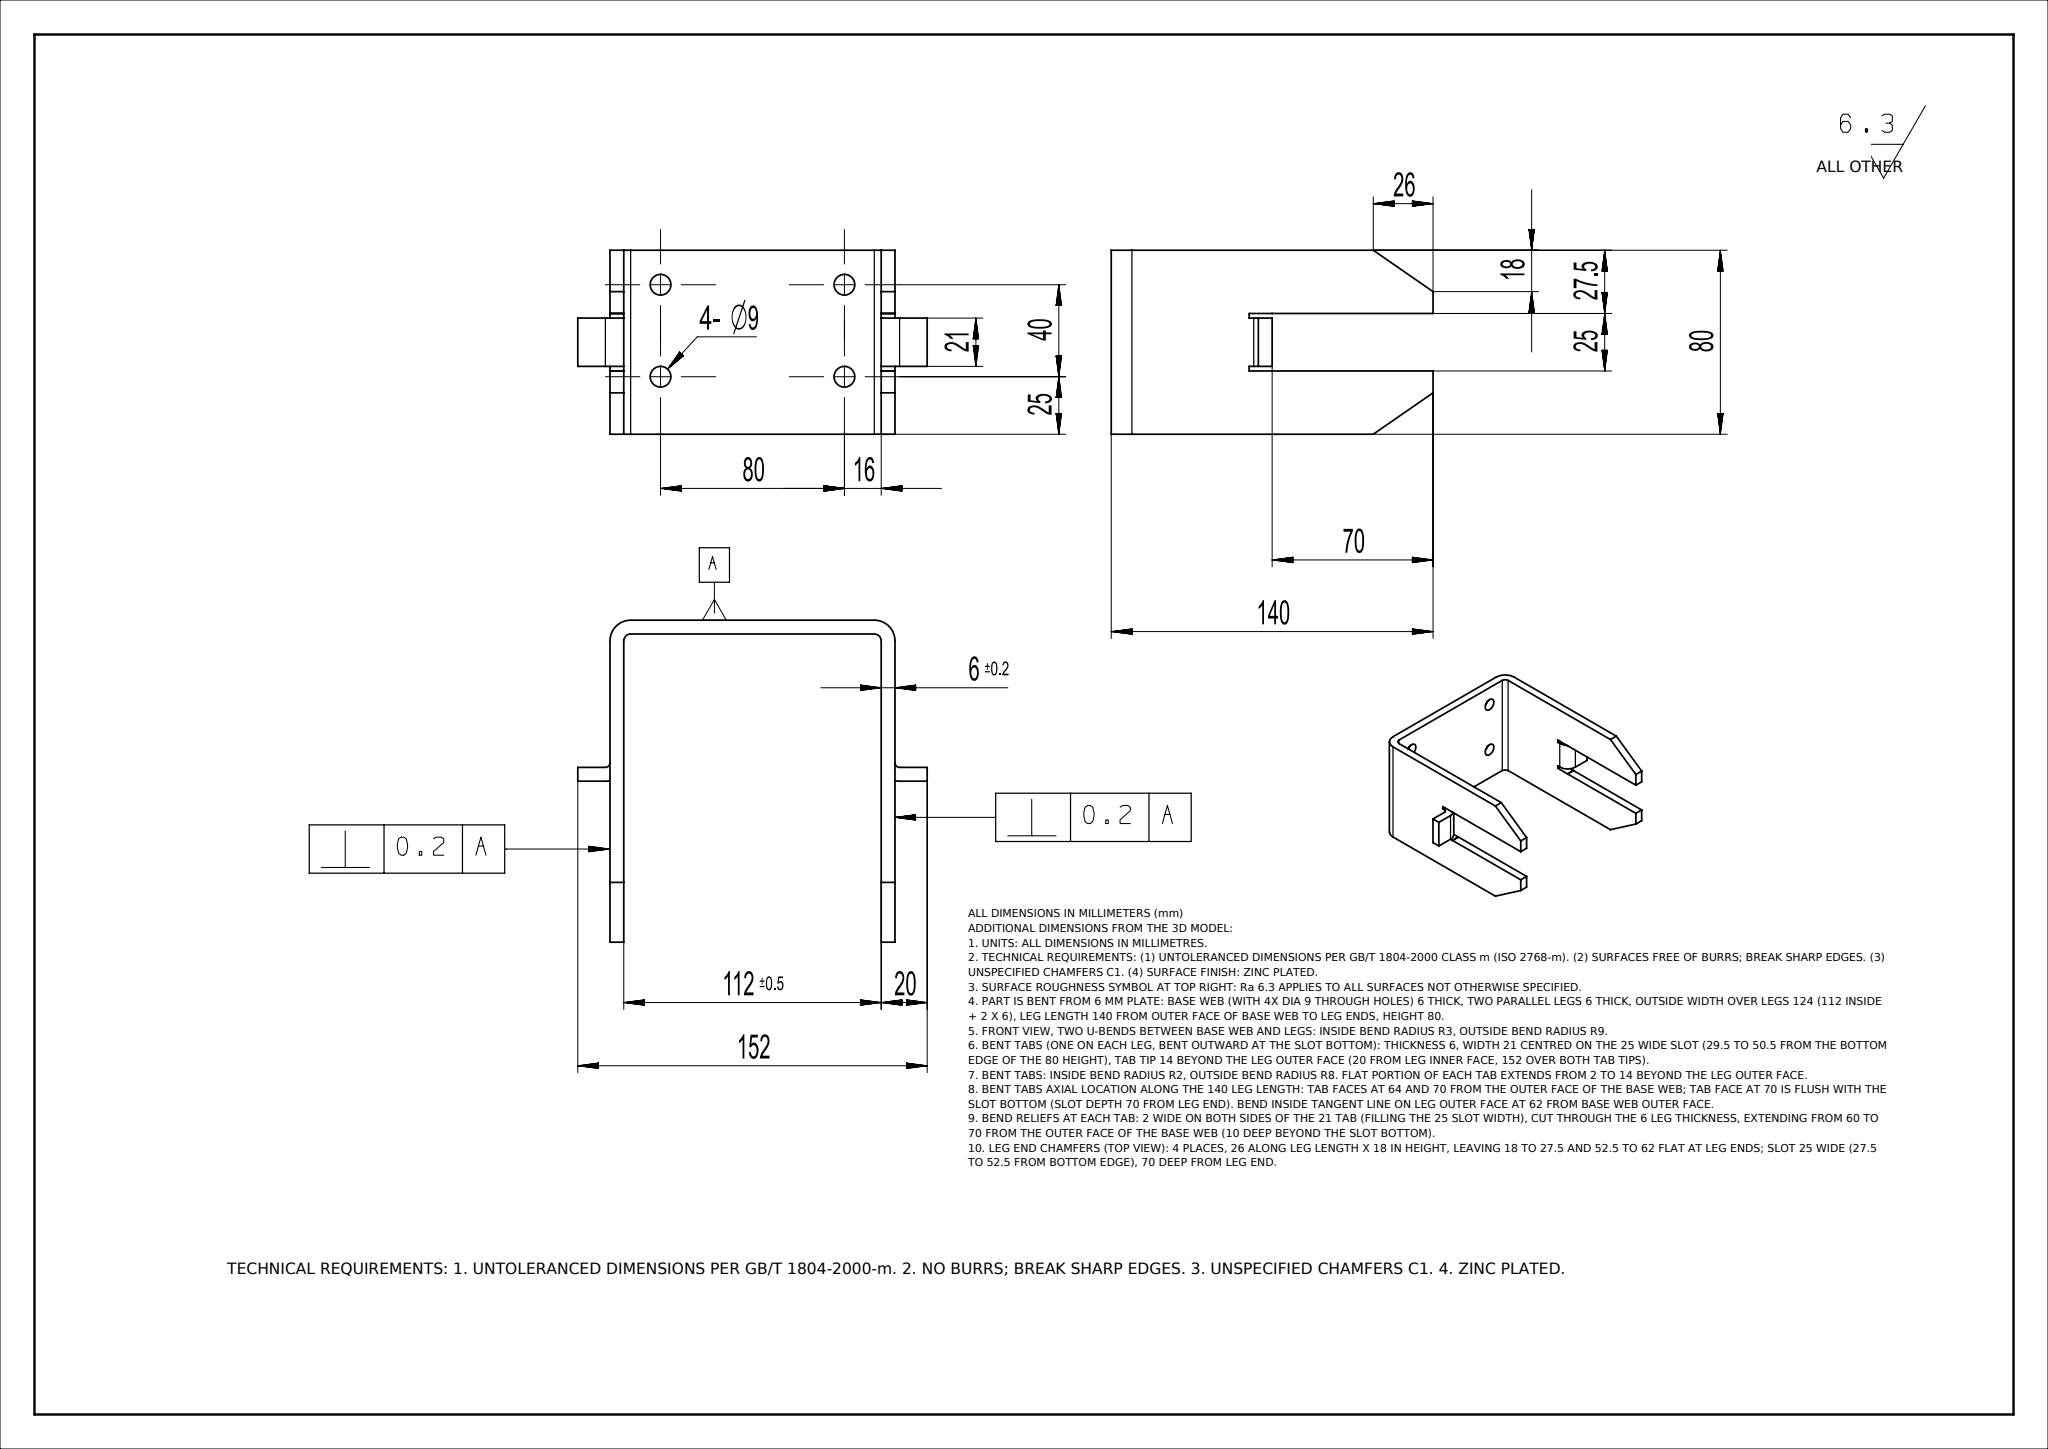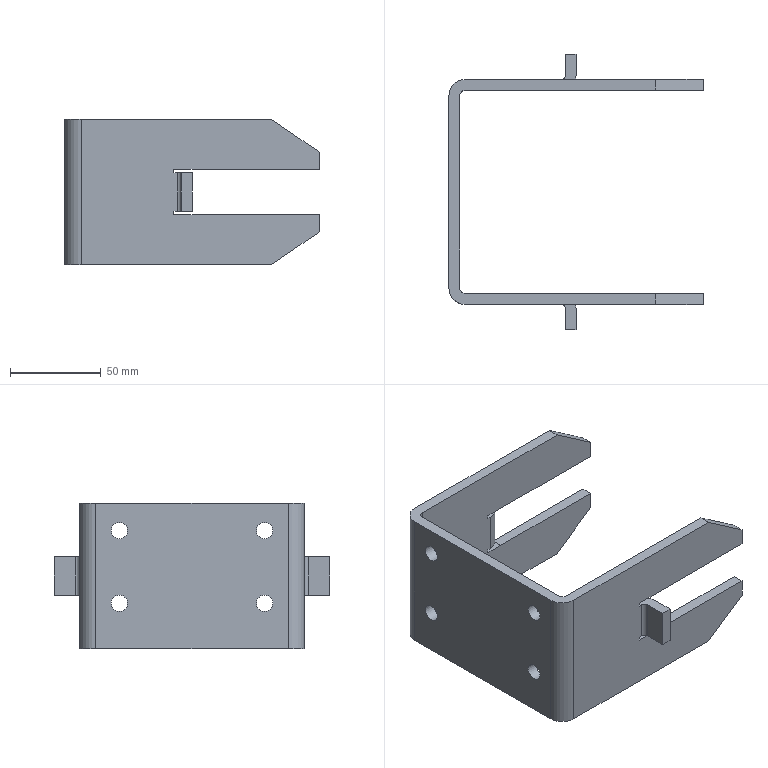Part | NX | mm | 1 solid | 54 faces | box 140 x 152 x 80 mm | volume 160052 mm3 | plane 42 | cylinder 12 | commonest cylinder face diameters 9 x4 6 x2 18 x2 16 x2 4 x2